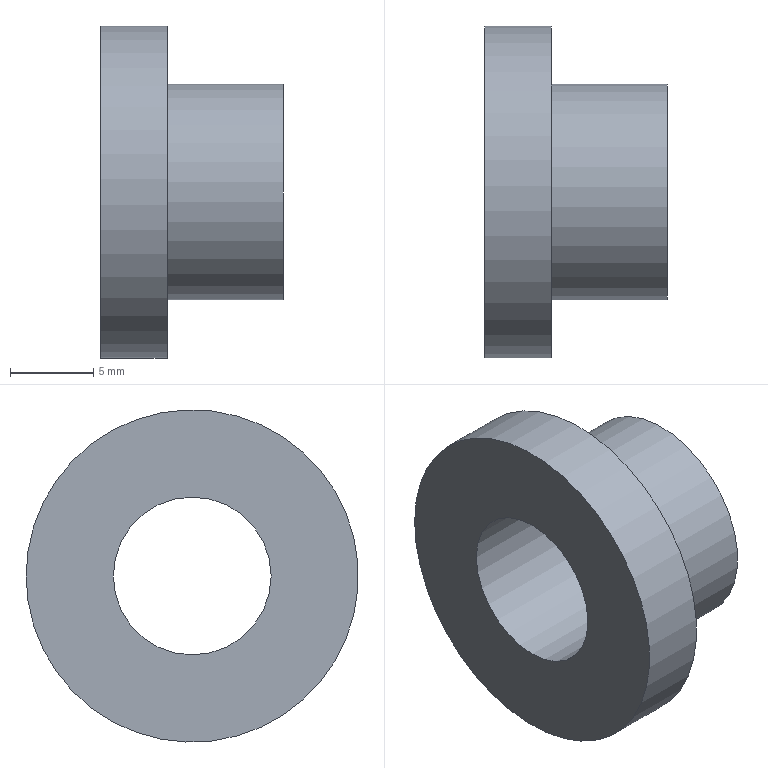Component | NX | BUSHING | 1 solid | 6 faces | box 11 x 20 x 20 mm | volume 1406 mm3 | plane 3 | cylinder 3 | commonest cylinder face diameters 13 x1 20 x1 9.5 x1
STEP:
#1=CARTESIAN_POINT('',(0.,0.,0.));
#2=DIRECTION('',(0.,0.,1.));
#3=DIRECTION('',(1.,0.,0.));
#4=AXIS2_PLACEMENT_3D('',#1,#2,#3);
#5=CARTESIAN_POINT('',(-155.,-4.75,255.5));
#6=VERTEX_POINT('',#5);
#7=CARTESIAN_POINT('',(-155.,4.75,255.5));
#8=VERTEX_POINT('',#7);
#9=CARTESIAN_POINT('',(-155.,-0.,255.5));
#10=DIRECTION('',(1.,0.,0.));
#11=DIRECTION('',(0.,-1.,0.));
#12=AXIS2_PLACEMENT_3D('',#9,#10,#11);
#13=CIRCLE('',#12,4.75);
#14=CARTESIAN_POINT('',(-155.,-0.,255.5));
#15=DIRECTION('',(1.,0.,0.));
#16=DIRECTION('',(0.,-1.,0.));
#17=AXIS2_PLACEMENT_3D('',#14,#15,#16);
#18=PLANE('',#17);
#19=CARTESIAN_POINT('',(0.,0.));
#20=DIRECTION('',(1.,0.));
#21=AXIS2_PLACEMENT_2D('',#19,#20);
#22=CIRCLE('',#21,4.75);
#23=(GEOMETRIC_REPRESENTATION_CONTEXT(2)PARAMETRIC_REPRESENTATION_CONTEXT()REPRESENTATION_CONTEXT('',''));
#24=DEFINITIONAL_REPRESENTATION('',(#22),#23);
#25=PCURVE('',#18,#24);
#26=CARTESIAN_POINT('',(-146.,-0.,255.5));
#27=DIRECTION('',(-1.,0.,0.));
#28=DIRECTION('',(0.,1.,0.));
#29=AXIS2_PLACEMENT_3D('',#26,#27,#28);
#30=CYLINDRICAL_SURFACE('',#29,4.75);
#31=CARTESIAN_POINT('',(3.142,9.));
#32=DIRECTION('',(-1.,0.));
#33=VECTOR('',#32,1.);
#34=LINE('',#31,#33);
#35=(GEOMETRIC_REPRESENTATION_CONTEXT(2)PARAMETRIC_REPRESENTATION_CONTEXT()REPRESENTATION_CONTEXT('',''));
#36=DEFINITIONAL_REPRESENTATION('',(#34),#35);
#37=PCURVE('',#30,#36);
#38=SURFACE_CURVE('',#13,(#25,#37),.PCURVE_S1.);
#39=EDGE_CURVE('',#6,#8,#38,.T.);
#40=ORIENTED_EDGE('',*,*,#39,.F.);
#41=CARTESIAN_POINT('',(-155.,-0.,255.5));
#42=DIRECTION('',(1.,0.,0.));
#43=DIRECTION('',(0.,-1.,0.));
#44=AXIS2_PLACEMENT_3D('',#41,#42,#43);
#45=CIRCLE('',#44,4.75);
#46=CARTESIAN_POINT('',(0.,0.));
#47=DIRECTION('',(1.,0.));
#48=AXIS2_PLACEMENT_2D('',#46,#47);
#49=CIRCLE('',#48,4.75);
#50=(GEOMETRIC_REPRESENTATION_CONTEXT(2)PARAMETRIC_REPRESENTATION_CONTEXT()REPRESENTATION_CONTEXT('',''));
#51=DEFINITIONAL_REPRESENTATION('',(#49),#50);
#52=PCURVE('',#18,#51);
#53=CARTESIAN_POINT('',(9.425,9.));
#54=DIRECTION('',(-1.,0.));
#55=VECTOR('',#54,1.);
#56=LINE('',#53,#55);
#57=(GEOMETRIC_REPRESENTATION_CONTEXT(2)PARAMETRIC_REPRESENTATION_CONTEXT()REPRESENTATION_CONTEXT('',''));
#58=DEFINITIONAL_REPRESENTATION('',(#56),#57);
#59=PCURVE('',#30,#58);
#60=SURFACE_CURVE('',#45,(#52,#59),.PCURVE_S1.);
#61=EDGE_CURVE('',#8,#6,#60,.T.);
#62=ORIENTED_EDGE('',*,*,#61,.F.);
#63=EDGE_LOOP('',(#40,#62));
#64=FACE_BOUND('',#63,.T.);
#65=CARTESIAN_POINT('',(-155.,6.5,255.5));
#66=VERTEX_POINT('',#65);
#67=CARTESIAN_POINT('',(-155.,-0.,255.5));
#68=DIRECTION('',(-1.,0.,0.));
#69=DIRECTION('',(0.,1.,0.));
#70=AXIS2_PLACEMENT_3D('',#67,#68,#69);
#71=CIRCLE('',#70,6.5);
#72=CARTESIAN_POINT('',(-6.5,0.));
#73=CARTESIAN_POINT('',(-6.5,11.258));
#74=CARTESIAN_POINT('',(3.25,5.629));
#75=CARTESIAN_POINT('',(13.,0.));
#76=CARTESIAN_POINT('',(3.25,-5.629));
#77=CARTESIAN_POINT('',(-6.5,-11.258));
#78=CARTESIAN_POINT('',(-6.5,0.));
#79=(BOUNDED_CURVE()B_SPLINE_CURVE(2,(#72,#73,#74,#75,#76,#77,#78),.UNSPECIFIED.,.T.,.F.)B_SPLINE_CURVE_WITH_KNOTS((1,2,2,2,2,1),(-2.094,0.,2.094,4.189,6.283,8.378),.UNSPECIFIED.)CURVE()GEOMETRIC_REPRESENTATION_ITEM()RATIONAL_B_SPLINE_CURVE((1.,0.5,1.,0.5,1.,0.5,1.))REPRESENTATION_ITEM(''));
#80=(GEOMETRIC_REPRESENTATION_CONTEXT(2)PARAMETRIC_REPRESENTATION_CONTEXT()REPRESENTATION_CONTEXT('',''));
#81=DEFINITIONAL_REPRESENTATION('',(#79),#80);
#82=PCURVE('',#18,#81);
#83=CARTESIAN_POINT('',(-155.,-0.,255.5));
#84=DIRECTION('',(-1.,0.,0.));
#85=DIRECTION('',(0.,1.,0.));
#86=AXIS2_PLACEMENT_3D('',#83,#84,#85);
#87=CYLINDRICAL_SURFACE('',#86,6.5);
#88=CARTESIAN_POINT('',(0.,0.));
#89=DIRECTION('',(1.,0.));
#90=VECTOR('',#89,1.);
#91=LINE('',#88,#90);
#92=(GEOMETRIC_REPRESENTATION_CONTEXT(2)PARAMETRIC_REPRESENTATION_CONTEXT()REPRESENTATION_CONTEXT('',''));
#93=DEFINITIONAL_REPRESENTATION('',(#91),#92);
#94=PCURVE('',#87,#93);
#95=SURFACE_CURVE('',#71,(#82,#94),.PCURVE_S1.);
#96=EDGE_CURVE('',#66,#66,#95,.T.);
#97=ORIENTED_EDGE('',*,*,#96,.F.);
#98=EDGE_LOOP('',(#97));
#99=FACE_BOUND('',#98,.T.);
#100=ADVANCED_FACE('',(#64,#99),#18,.T.);
#101=CARTESIAN_POINT('',(-162.,6.5,255.5));
#102=VERTEX_POINT('',#101);
#103=CARTESIAN_POINT('',(-162.,-0.,255.5));
#104=DIRECTION('',(1.,0.,0.));
#105=DIRECTION('',(0.,1.,0.));
#106=AXIS2_PLACEMENT_3D('',#103,#104,#105);
#107=CIRCLE('',#106,6.5);
#108=CARTESIAN_POINT('',(6.283,7.));
#109=DIRECTION('',(-1.,0.));
#110=VECTOR('',#109,1.);
#111=LINE('',#108,#110);
#112=(GEOMETRIC_REPRESENTATION_CONTEXT(2)PARAMETRIC_REPRESENTATION_CONTEXT()REPRESENTATION_CONTEXT('',''));
#113=DEFINITIONAL_REPRESENTATION('',(#111),#112);
#114=PCURVE('',#87,#113);
#115=CARTESIAN_POINT('',(-162.,-0.,255.5));
#116=DIRECTION('',(1.,0.,0.));
#117=DIRECTION('',(0.,-1.,0.));
#118=AXIS2_PLACEMENT_3D('',#115,#116,#117);
#119=PLANE('',#118);
#120=CARTESIAN_POINT('',(0.,0.));
#121=DIRECTION('',(-1.,0.));
#122=AXIS2_PLACEMENT_2D('',#120,#121);
#123=CIRCLE('',#122,6.5);
#124=(GEOMETRIC_REPRESENTATION_CONTEXT(2)PARAMETRIC_REPRESENTATION_CONTEXT()REPRESENTATION_CONTEXT('',''));
#125=DEFINITIONAL_REPRESENTATION('',(#123),#124);
#126=PCURVE('',#119,#125);
#127=SURFACE_CURVE('',#107,(#114,#126),.PCURVE_S1.);
#128=EDGE_CURVE('',#102,#102,#127,.T.);
#129=ORIENTED_EDGE('',*,*,#128,.T.);
#130=CARTESIAN_POINT('',(-155.,6.5,255.5));
#131=CARTESIAN_POINT('',(-162.,6.5,255.5));
#132=B_SPLINE_CURVE_WITH_KNOTS('',1,(#130,#131),.UNSPECIFIED.,.F.,.F.,(2,2),(0.,7.),.PIECEWISE_BEZIER_KNOTS.);
#133=CARTESIAN_POINT('',(0.,0.));
#134=DIRECTION('',(0.,1.));
#135=VECTOR('',#134,1.);
#136=LINE('',#133,#135);
#137=(GEOMETRIC_REPRESENTATION_CONTEXT(2)PARAMETRIC_REPRESENTATION_CONTEXT()REPRESENTATION_CONTEXT('',''));
#138=DEFINITIONAL_REPRESENTATION('',(#136),#137);
#139=PCURVE('',#87,#138);
#140=CARTESIAN_POINT('',(6.283,0.));
#141=DIRECTION('',(0.,1.));
#142=VECTOR('',#141,1.);
#143=LINE('',#140,#142);
#144=(GEOMETRIC_REPRESENTATION_CONTEXT(2)PARAMETRIC_REPRESENTATION_CONTEXT()REPRESENTATION_CONTEXT('',''));
#145=DEFINITIONAL_REPRESENTATION('',(#143),#144);
#146=PCURVE('',#87,#145);
#147=SEAM_CURVE('',#132,(#139,#146),.PCURVE_S1.);
#148=EDGE_CURVE('',#66,#102,#147,.T.);
#149=ORIENTED_EDGE('',*,*,#148,.F.);
#150=ORIENTED_EDGE('',*,*,#96,.T.);
#151=ORIENTED_EDGE('',*,*,#148,.T.);
#152=EDGE_LOOP('',(#129,#149,#150,#151));
#153=FACE_BOUND('',#152,.T.);
#154=ADVANCED_FACE('',(#153),#87,.T.);
#155=CARTESIAN_POINT('',(-166.,4.75,255.5));
#156=VERTEX_POINT('',#155);
#157=CARTESIAN_POINT('',(-166.,-0.,255.5));
#158=DIRECTION('',(-1.,0.,0.));
#159=DIRECTION('',(0.,1.,0.));
#160=AXIS2_PLACEMENT_3D('',#157,#158,#159);
#161=CIRCLE('',#160,4.75);
#162=CARTESIAN_POINT('',(-166.,-0.,255.5));
#163=DIRECTION('',(-1.,0.,0.));
#164=DIRECTION('',(0.,1.,0.));
#165=AXIS2_PLACEMENT_3D('',#162,#163,#164);
#166=PLANE('',#165);
#167=CARTESIAN_POINT('',(0.,0.));
#168=DIRECTION('',(1.,0.));
#169=AXIS2_PLACEMENT_2D('',#167,#168);
#170=CIRCLE('',#169,4.75);
#171=(GEOMETRIC_REPRESENTATION_CONTEXT(2)PARAMETRIC_REPRESENTATION_CONTEXT()REPRESENTATION_CONTEXT('',''));
#172=DEFINITIONAL_REPRESENTATION('',(#170),#171);
#173=PCURVE('',#166,#172);
#174=CARTESIAN_POINT('',(0.,20.));
#175=DIRECTION('',(1.,0.));
#176=VECTOR('',#175,1.);
#177=LINE('',#174,#176);
#178=(GEOMETRIC_REPRESENTATION_CONTEXT(2)PARAMETRIC_REPRESENTATION_CONTEXT()REPRESENTATION_CONTEXT('',''));
#179=DEFINITIONAL_REPRESENTATION('',(#177),#178);
#180=PCURVE('',#30,#179);
#181=SURFACE_CURVE('',#161,(#173,#180),.PCURVE_S1.);
#182=EDGE_CURVE('',#156,#156,#181,.T.);
#183=ORIENTED_EDGE('',*,*,#182,.F.);
#184=EDGE_LOOP('',(#183));
#185=FACE_BOUND('',#184,.T.);
#186=CARTESIAN_POINT('',(-166.,10.,255.5));
#187=VERTEX_POINT('',#186);
#188=CARTESIAN_POINT('',(-166.,-0.,255.5));
#189=DIRECTION('',(-1.,0.,0.));
#190=DIRECTION('',(0.,1.,0.));
#191=AXIS2_PLACEMENT_3D('',#188,#189,#190);
#192=CIRCLE('',#191,10.);
#193=CARTESIAN_POINT('',(0.,0.));
#194=DIRECTION('',(1.,0.));
#195=AXIS2_PLACEMENT_2D('',#193,#194);
#196=CIRCLE('',#195,10.);
#197=(GEOMETRIC_REPRESENTATION_CONTEXT(2)PARAMETRIC_REPRESENTATION_CONTEXT()REPRESENTATION_CONTEXT('',''));
#198=DEFINITIONAL_REPRESENTATION('',(#196),#197);
#199=PCURVE('',#166,#198);
#200=CARTESIAN_POINT('',(-162.,-0.,255.5));
#201=DIRECTION('',(-1.,0.,0.));
#202=DIRECTION('',(0.,1.,0.));
#203=AXIS2_PLACEMENT_3D('',#200,#201,#202);
#204=CYLINDRICAL_SURFACE('',#203,10.);
#205=CARTESIAN_POINT('',(0.,4.));
#206=DIRECTION('',(1.,0.));
#207=VECTOR('',#206,1.);
#208=LINE('',#205,#207);
#209=(GEOMETRIC_REPRESENTATION_CONTEXT(2)PARAMETRIC_REPRESENTATION_CONTEXT()REPRESENTATION_CONTEXT('',''));
#210=DEFINITIONAL_REPRESENTATION('',(#208),#209);
#211=PCURVE('',#204,#210);
#212=SURFACE_CURVE('',#192,(#199,#211),.PCURVE_S1.);
#213=EDGE_CURVE('',#187,#187,#212,.T.);
#214=ORIENTED_EDGE('',*,*,#213,.T.);
#215=EDGE_LOOP('',(#214));
#216=FACE_BOUND('',#215,.T.);
#217=ADVANCED_FACE('',(#185,#216),#166,.T.);
#218=ORIENTED_EDGE('',*,*,#128,.F.);
#219=EDGE_LOOP('',(#218));
#220=FACE_BOUND('',#219,.T.);
#221=CARTESIAN_POINT('',(-162.,10.,255.5));
#222=VERTEX_POINT('',#221);
#223=CARTESIAN_POINT('',(-162.,-0.,255.5));
#224=DIRECTION('',(-1.,0.,0.));
#225=DIRECTION('',(0.,1.,0.));
#226=AXIS2_PLACEMENT_3D('',#223,#224,#225);
#227=CIRCLE('',#226,10.);
#228=CARTESIAN_POINT('',(-10.,0.));
#229=CARTESIAN_POINT('',(-10.,17.321));
#230=CARTESIAN_POINT('',(5.,8.66));
#231=CARTESIAN_POINT('',(20.,0.));
#232=CARTESIAN_POINT('',(5.,-8.66));
#233=CARTESIAN_POINT('',(-10.,-17.321));
#234=CARTESIAN_POINT('',(-10.,0.));
#235=(BOUNDED_CURVE()B_SPLINE_CURVE(2,(#228,#229,#230,#231,#232,#233,#234),.UNSPECIFIED.,.T.,.F.)B_SPLINE_CURVE_WITH_KNOTS((1,2,2,2,2,1),(-2.094,0.,2.094,4.189,6.283,8.378),.UNSPECIFIED.)CURVE()GEOMETRIC_REPRESENTATION_ITEM()RATIONAL_B_SPLINE_CURVE((1.,0.5,1.,0.5,1.,0.5,1.))REPRESENTATION_ITEM(''));
#236=(GEOMETRIC_REPRESENTATION_CONTEXT(2)PARAMETRIC_REPRESENTATION_CONTEXT()REPRESENTATION_CONTEXT('',''));
#237=DEFINITIONAL_REPRESENTATION('',(#235),#236);
#238=PCURVE('',#119,#237);
#239=CARTESIAN_POINT('',(0.,0.));
#240=DIRECTION('',(1.,0.));
#241=VECTOR('',#240,1.);
#242=LINE('',#239,#241);
#243=(GEOMETRIC_REPRESENTATION_CONTEXT(2)PARAMETRIC_REPRESENTATION_CONTEXT()REPRESENTATION_CONTEXT('',''));
#244=DEFINITIONAL_REPRESENTATION('',(#242),#243);
#245=PCURVE('',#204,#244);
#246=SURFACE_CURVE('',#227,(#238,#245),.PCURVE_S1.);
#247=EDGE_CURVE('',#222,#222,#246,.T.);
#248=ORIENTED_EDGE('',*,*,#247,.F.);
#249=EDGE_LOOP('',(#248));
#250=FACE_BOUND('',#249,.T.);
#251=ADVANCED_FACE('',(#220,#250),#119,.T.);
#252=ORIENTED_EDGE('',*,*,#213,.F.);
#253=CARTESIAN_POINT('',(-162.,10.,255.5));
#254=CARTESIAN_POINT('',(-166.,10.,255.5));
#255=B_SPLINE_CURVE_WITH_KNOTS('',1,(#253,#254),.UNSPECIFIED.,.F.,.F.,(2,2),(0.,4.),.PIECEWISE_BEZIER_KNOTS.);
#256=CARTESIAN_POINT('',(0.,0.));
#257=DIRECTION('',(0.,1.));
#258=VECTOR('',#257,1.);
#259=LINE('',#256,#258);
#260=(GEOMETRIC_REPRESENTATION_CONTEXT(2)PARAMETRIC_REPRESENTATION_CONTEXT()REPRESENTATION_CONTEXT('',''));
#261=DEFINITIONAL_REPRESENTATION('',(#259),#260);
#262=PCURVE('',#204,#261);
#263=CARTESIAN_POINT('',(6.283,0.));
#264=DIRECTION('',(0.,1.));
#265=VECTOR('',#264,1.);
#266=LINE('',#263,#265);
#267=(GEOMETRIC_REPRESENTATION_CONTEXT(2)PARAMETRIC_REPRESENTATION_CONTEXT()REPRESENTATION_CONTEXT('',''));
#268=DEFINITIONAL_REPRESENTATION('',(#266),#267);
#269=PCURVE('',#204,#268);
#270=SEAM_CURVE('',#255,(#262,#269),.PCURVE_S1.);
#271=EDGE_CURVE('',#222,#187,#270,.T.);
#272=ORIENTED_EDGE('',*,*,#271,.F.);
#273=ORIENTED_EDGE('',*,*,#247,.T.);
#274=ORIENTED_EDGE('',*,*,#271,.T.);
#275=EDGE_LOOP('',(#252,#272,#273,#274));
#276=FACE_BOUND('',#275,.T.);
#277=ADVANCED_FACE('',(#276),#204,.T.);
#278=ORIENTED_EDGE('',*,*,#61,.F.);
#279=CARTESIAN_POINT('',(-155.,4.75,255.5));
#280=CARTESIAN_POINT('',(-166.,4.75,255.5));
#281=B_SPLINE_CURVE_WITH_KNOTS('',1,(#279,#280),.UNSPECIFIED.,.F.,.F.,(2,2),(9.,20.),.PIECEWISE_BEZIER_KNOTS.);
#282=CARTESIAN_POINT('',(6.283,0.));
#283=DIRECTION('',(0.,1.));
#284=VECTOR('',#283,1.);
#285=LINE('',#282,#284);
#286=(GEOMETRIC_REPRESENTATION_CONTEXT(2)PARAMETRIC_REPRESENTATION_CONTEXT()REPRESENTATION_CONTEXT('',''));
#287=DEFINITIONAL_REPRESENTATION('',(#285),#286);
#288=PCURVE('',#30,#287);
#289=CARTESIAN_POINT('',(0.,0.));
#290=DIRECTION('',(0.,1.));
#291=VECTOR('',#290,1.);
#292=LINE('',#289,#291);
#293=(GEOMETRIC_REPRESENTATION_CONTEXT(2)PARAMETRIC_REPRESENTATION_CONTEXT()REPRESENTATION_CONTEXT('',''));
#294=DEFINITIONAL_REPRESENTATION('',(#292),#293);
#295=PCURVE('',#30,#294);
#296=SEAM_CURVE('',#281,(#288,#295),.PCURVE_S1.);
#297=EDGE_CURVE('',#8,#156,#296,.T.);
#298=ORIENTED_EDGE('',*,*,#297,.T.);
#299=ORIENTED_EDGE('',*,*,#182,.F.);
#300=ORIENTED_EDGE('',*,*,#297,.F.);
#301=ORIENTED_EDGE('',*,*,#39,.F.);
#302=EDGE_LOOP('',(#278,#298,#299,#300,#301));
#303=FACE_BOUND('',#302,.F.);
#304=ADVANCED_FACE('',(#303),#30,.F.);
#305=CLOSED_SHELL('',(#100,#154,#217,#251,#277,#304));
#306=MANIFOLD_SOLID_BREP('',#305);
#307=(LENGTH_UNIT()NAMED_UNIT(*)SI_UNIT(.MILLI.,.METRE.));
#308=UNCERTAINTY_MEASURE_WITH_UNIT(LENGTH_MEASURE(0.000005),#307,'','');
#309=(NAMED_UNIT(*)PLANE_ANGLE_UNIT()SI_UNIT($,.RADIAN.));
#310=(NAMED_UNIT(*)SI_UNIT($,.STERADIAN.)SOLID_ANGLE_UNIT());
#311=(GEOMETRIC_REPRESENTATION_CONTEXT(3)GLOBAL_UNCERTAINTY_ASSIGNED_CONTEXT((#308))GLOBAL_UNIT_ASSIGNED_CONTEXT((#307,#309,#310))REPRESENTATION_CONTEXT('',''));
#312=ADVANCED_BREP_SHAPE_REPRESENTATION('',(#4,#306),#311);